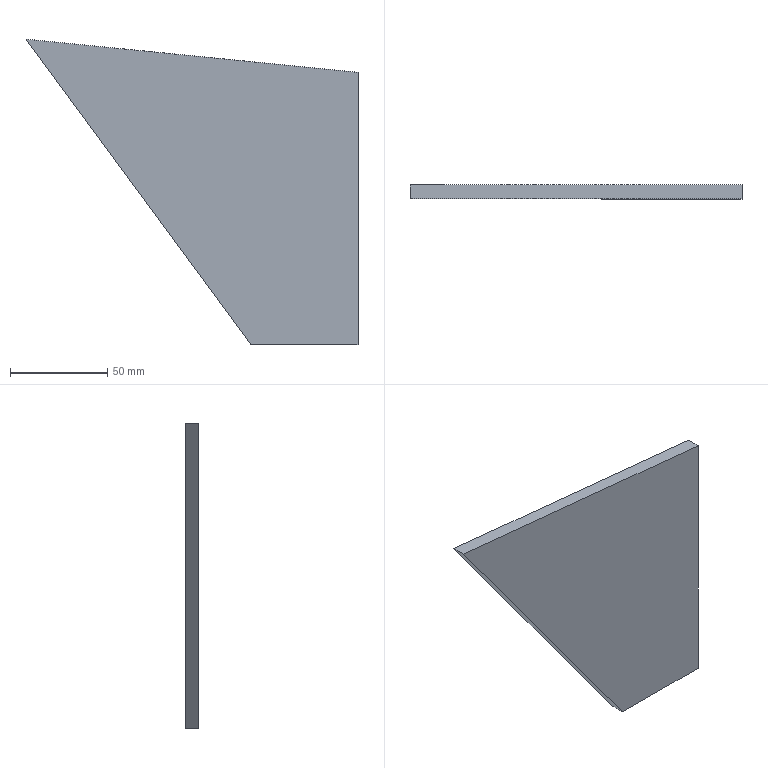Component | NX | TRIANGLE1_3 | 1 solid | 6 faces | box 170.57 x 7 x 157.02 mm | volume 113806 mm3 | plane 6
STEP:
#1=CARTESIAN_POINT('',(0.,0.,0.));
#2=DIRECTION('',(0.,0.,1.));
#3=DIRECTION('',(1.,0.,0.));
#4=AXIS2_PLACEMENT_3D('',#1,#2,#3);
#5=CARTESIAN_POINT('',(0.,142.,371.782));
#6=VERTEX_POINT('',#5);
#7=CARTESIAN_POINT('',(-115.568,142.,528.807));
#8=VERTEX_POINT('',#7);
#9=CARTESIAN_POINT('',(0.,142.,371.782));
#10=DIRECTION('',(-0.5928,0.,0.8054));
#11=VECTOR('',#10,1.);
#12=LINE('',#9,#11);
#13=CARTESIAN_POINT('',(0.,135.,371.782));
#14=DIRECTION('',(-0.8054,0.,-0.5928));
#15=DIRECTION('',(-0.5928,0.,0.8054));
#16=AXIS2_PLACEMENT_3D('',#13,#14,#15);
#17=PLANE('',#16);
#18=CARTESIAN_POINT('',(0.,7.));
#19=DIRECTION('',(1.,0.));
#20=VECTOR('',#19,1.);
#21=LINE('',#18,#20);
#22=(GEOMETRIC_REPRESENTATION_CONTEXT(2)PARAMETRIC_REPRESENTATION_CONTEXT()REPRESENTATION_CONTEXT('',''));
#23=DEFINITIONAL_REPRESENTATION('',(#21),#22);
#24=PCURVE('',#17,#23);
#25=CARTESIAN_POINT('',(-0.,142.,371.782));
#26=DIRECTION('',(0.,-1.,0.));
#27=DIRECTION('',(0.,0.,-1.));
#28=AXIS2_PLACEMENT_3D('',#25,#26,#27);
#29=PLANE('',#28);
#30=CARTESIAN_POINT('',(0.,0.));
#31=DIRECTION('',(-0.8054,-0.5928));
#32=VECTOR('',#31,1.);
#33=LINE('',#30,#32);
#34=(GEOMETRIC_REPRESENTATION_CONTEXT(2)PARAMETRIC_REPRESENTATION_CONTEXT()REPRESENTATION_CONTEXT('',''));
#35=DEFINITIONAL_REPRESENTATION('',(#33),#34);
#36=PCURVE('',#29,#35);
#37=SURFACE_CURVE('',#12,(#24,#36),.PCURVE_S1.);
#38=EDGE_CURVE('',#6,#8,#37,.T.);
#39=ORIENTED_EDGE('',*,*,#38,.F.);
#40=CARTESIAN_POINT('',(0.,135.,371.782));
#41=VERTEX_POINT('',#40);
#42=CARTESIAN_POINT('',(0.,135.,371.782));
#43=DIRECTION('',(0.,1.,0.));
#44=VECTOR('',#43,1.);
#45=LINE('',#42,#44);
#46=CARTESIAN_POINT('',(0.,0.));
#47=DIRECTION('',(0.,1.));
#48=VECTOR('',#47,1.);
#49=LINE('',#46,#48);
#50=(GEOMETRIC_REPRESENTATION_CONTEXT(2)PARAMETRIC_REPRESENTATION_CONTEXT()REPRESENTATION_CONTEXT('',''));
#51=DEFINITIONAL_REPRESENTATION('',(#49),#50);
#52=PCURVE('',#17,#51);
#53=CARTESIAN_POINT('',(55.,135.,371.782));
#54=DIRECTION('',(-0.,0.,-1.));
#55=DIRECTION('',(-1.,0.,0.));
#56=AXIS2_PLACEMENT_3D('',#53,#54,#55);
#57=PLANE('',#56);
#58=CARTESIAN_POINT('',(55.,0.));
#59=DIRECTION('',(0.,1.));
#60=VECTOR('',#59,1.);
#61=LINE('',#58,#60);
#62=(GEOMETRIC_REPRESENTATION_CONTEXT(2)PARAMETRIC_REPRESENTATION_CONTEXT()REPRESENTATION_CONTEXT('',''));
#63=DEFINITIONAL_REPRESENTATION('',(#61),#62);
#64=PCURVE('',#57,#63);
#65=SURFACE_CURVE('',#45,(#52,#64),.PCURVE_S1.);
#66=EDGE_CURVE('',#41,#6,#65,.T.);
#67=ORIENTED_EDGE('',*,*,#66,.F.);
#68=CARTESIAN_POINT('',(-115.568,135.,528.807));
#69=VERTEX_POINT('',#68);
#70=CARTESIAN_POINT('',(0.,135.,371.782));
#71=DIRECTION('',(-0.5928,0.,0.8054));
#72=VECTOR('',#71,1.);
#73=LINE('',#70,#72);
#74=CARTESIAN_POINT('',(0.,0.));
#75=DIRECTION('',(1.,0.));
#76=VECTOR('',#75,1.);
#77=LINE('',#74,#76);
#78=(GEOMETRIC_REPRESENTATION_CONTEXT(2)PARAMETRIC_REPRESENTATION_CONTEXT()REPRESENTATION_CONTEXT('',''));
#79=DEFINITIONAL_REPRESENTATION('',(#77),#78);
#80=PCURVE('',#17,#79);
#81=CARTESIAN_POINT('',(-0.,135.,371.782));
#82=DIRECTION('',(0.,-1.,0.));
#83=DIRECTION('',(0.,0.,-1.));
#84=AXIS2_PLACEMENT_3D('',#81,#82,#83);
#85=PLANE('',#84);
#86=CARTESIAN_POINT('',(0.,0.));
#87=DIRECTION('',(-0.8054,-0.5928));
#88=VECTOR('',#87,1.);
#89=LINE('',#86,#88);
#90=(GEOMETRIC_REPRESENTATION_CONTEXT(2)PARAMETRIC_REPRESENTATION_CONTEXT()REPRESENTATION_CONTEXT('',''));
#91=DEFINITIONAL_REPRESENTATION('',(#89),#90);
#92=PCURVE('',#85,#91);
#93=SURFACE_CURVE('',#73,(#80,#92),.PCURVE_S1.);
#94=EDGE_CURVE('',#41,#69,#93,.T.);
#95=ORIENTED_EDGE('',*,*,#94,.T.);
#96=CARTESIAN_POINT('',(-115.568,135.,528.807));
#97=DIRECTION('',(0.,1.,0.));
#98=VECTOR('',#97,1.);
#99=LINE('',#96,#98);
#100=CARTESIAN_POINT('',(194.969,0.));
#101=DIRECTION('',(0.,1.));
#102=VECTOR('',#101,1.);
#103=LINE('',#100,#102);
#104=(GEOMETRIC_REPRESENTATION_CONTEXT(2)PARAMETRIC_REPRESENTATION_CONTEXT()REPRESENTATION_CONTEXT('',''));
#105=DEFINITIONAL_REPRESENTATION('',(#103),#104);
#106=PCURVE('',#17,#105);
#107=CARTESIAN_POINT('',(-115.568,135.,528.807));
#108=DIRECTION('',(0.09932,0.,0.9951));
#109=DIRECTION('',(0.9951,0.,-0.09932));
#110=AXIS2_PLACEMENT_3D('',#107,#108,#109);
#111=PLANE('',#110);
#112=CARTESIAN_POINT('',(0.,0.));
#113=DIRECTION('',(0.,1.));
#114=VECTOR('',#113,1.);
#115=LINE('',#112,#114);
#116=(GEOMETRIC_REPRESENTATION_CONTEXT(2)PARAMETRIC_REPRESENTATION_CONTEXT()REPRESENTATION_CONTEXT('',''));
#117=DEFINITIONAL_REPRESENTATION('',(#115),#116);
#118=PCURVE('',#111,#117);
#119=SURFACE_CURVE('',#99,(#106,#118),.PCURVE_S1.);
#120=EDGE_CURVE('',#69,#8,#119,.T.);
#121=ORIENTED_EDGE('',*,*,#120,.T.);
#122=EDGE_LOOP('',(#39,#67,#95,#121));
#123=FACE_BOUND('',#122,.T.);
#124=ADVANCED_FACE('',(#123),#17,.T.);
#125=CARTESIAN_POINT('',(55.,142.,511.782));
#126=VERTEX_POINT('',#125);
#127=CARTESIAN_POINT('',(-115.568,142.,528.807));
#128=DIRECTION('',(0.9951,0.,-0.09932));
#129=VECTOR('',#128,1.);
#130=LINE('',#127,#129);
#131=CARTESIAN_POINT('',(0.,7.));
#132=DIRECTION('',(1.,0.));
#133=VECTOR('',#132,1.);
#134=LINE('',#131,#133);
#135=(GEOMETRIC_REPRESENTATION_CONTEXT(2)PARAMETRIC_REPRESENTATION_CONTEXT()REPRESENTATION_CONTEXT('',''));
#136=DEFINITIONAL_REPRESENTATION('',(#134),#135);
#137=PCURVE('',#111,#136);
#138=CARTESIAN_POINT('',(-157.025,-115.568));
#139=DIRECTION('',(0.09932,0.9951));
#140=VECTOR('',#139,1.);
#141=LINE('',#138,#140);
#142=(GEOMETRIC_REPRESENTATION_CONTEXT(2)PARAMETRIC_REPRESENTATION_CONTEXT()REPRESENTATION_CONTEXT('',''));
#143=DEFINITIONAL_REPRESENTATION('',(#141),#142);
#144=PCURVE('',#29,#143);
#145=SURFACE_CURVE('',#130,(#137,#144),.PCURVE_S1.);
#146=EDGE_CURVE('',#8,#126,#145,.T.);
#147=ORIENTED_EDGE('',*,*,#146,.F.);
#148=ORIENTED_EDGE('',*,*,#120,.F.);
#149=CARTESIAN_POINT('',(55.,135.,511.782));
#150=VERTEX_POINT('',#149);
#151=CARTESIAN_POINT('',(-115.568,135.,528.807));
#152=DIRECTION('',(0.9951,0.,-0.09932));
#153=VECTOR('',#152,1.);
#154=LINE('',#151,#153);
#155=CARTESIAN_POINT('',(0.,0.));
#156=DIRECTION('',(1.,0.));
#157=VECTOR('',#156,1.);
#158=LINE('',#155,#157);
#159=(GEOMETRIC_REPRESENTATION_CONTEXT(2)PARAMETRIC_REPRESENTATION_CONTEXT()REPRESENTATION_CONTEXT('',''));
#160=DEFINITIONAL_REPRESENTATION('',(#158),#159);
#161=PCURVE('',#111,#160);
#162=CARTESIAN_POINT('',(-157.025,-115.568));
#163=DIRECTION('',(0.09932,0.9951));
#164=VECTOR('',#163,1.);
#165=LINE('',#162,#164);
#166=(GEOMETRIC_REPRESENTATION_CONTEXT(2)PARAMETRIC_REPRESENTATION_CONTEXT()REPRESENTATION_CONTEXT('',''));
#167=DEFINITIONAL_REPRESENTATION('',(#165),#166);
#168=PCURVE('',#85,#167);
#169=SURFACE_CURVE('',#154,(#161,#168),.PCURVE_S1.);
#170=EDGE_CURVE('',#69,#150,#169,.T.);
#171=ORIENTED_EDGE('',*,*,#170,.T.);
#172=CARTESIAN_POINT('',(55.,135.,511.782));
#173=DIRECTION('',(0.,1.,0.));
#174=VECTOR('',#173,1.);
#175=LINE('',#172,#174);
#176=CARTESIAN_POINT('',(171.415,0.));
#177=DIRECTION('',(0.,1.));
#178=VECTOR('',#177,1.);
#179=LINE('',#176,#178);
#180=(GEOMETRIC_REPRESENTATION_CONTEXT(2)PARAMETRIC_REPRESENTATION_CONTEXT()REPRESENTATION_CONTEXT('',''));
#181=DEFINITIONAL_REPRESENTATION('',(#179),#180);
#182=PCURVE('',#111,#181);
#183=CARTESIAN_POINT('',(55.,135.,511.782));
#184=DIRECTION('',(1.,0.,0.));
#185=DIRECTION('',(0.,0.,-1.));
#186=AXIS2_PLACEMENT_3D('',#183,#184,#185);
#187=PLANE('',#186);
#188=CARTESIAN_POINT('',(0.,0.));
#189=DIRECTION('',(0.,1.));
#190=VECTOR('',#189,1.);
#191=LINE('',#188,#190);
#192=(GEOMETRIC_REPRESENTATION_CONTEXT(2)PARAMETRIC_REPRESENTATION_CONTEXT()REPRESENTATION_CONTEXT('',''));
#193=DEFINITIONAL_REPRESENTATION('',(#191),#192);
#194=PCURVE('',#187,#193);
#195=SURFACE_CURVE('',#175,(#182,#194),.PCURVE_S1.);
#196=EDGE_CURVE('',#150,#126,#195,.T.);
#197=ORIENTED_EDGE('',*,*,#196,.T.);
#198=EDGE_LOOP('',(#147,#148,#171,#197));
#199=FACE_BOUND('',#198,.T.);
#200=ADVANCED_FACE('',(#199),#111,.T.);
#201=CARTESIAN_POINT('',(55.,142.,371.782));
#202=VERTEX_POINT('',#201);
#203=CARTESIAN_POINT('',(55.,142.,511.782));
#204=DIRECTION('',(0.,0.,-1.));
#205=VECTOR('',#204,1.);
#206=LINE('',#203,#205);
#207=CARTESIAN_POINT('',(0.,7.));
#208=DIRECTION('',(1.,0.));
#209=VECTOR('',#208,1.);
#210=LINE('',#207,#209);
#211=(GEOMETRIC_REPRESENTATION_CONTEXT(2)PARAMETRIC_REPRESENTATION_CONTEXT()REPRESENTATION_CONTEXT('',''));
#212=DEFINITIONAL_REPRESENTATION('',(#210),#211);
#213=PCURVE('',#187,#212);
#214=CARTESIAN_POINT('',(-140.,55.));
#215=DIRECTION('',(1.,0.));
#216=VECTOR('',#215,1.);
#217=LINE('',#214,#216);
#218=(GEOMETRIC_REPRESENTATION_CONTEXT(2)PARAMETRIC_REPRESENTATION_CONTEXT()REPRESENTATION_CONTEXT('',''));
#219=DEFINITIONAL_REPRESENTATION('',(#217),#218);
#220=PCURVE('',#29,#219);
#221=SURFACE_CURVE('',#206,(#213,#220),.PCURVE_S1.);
#222=EDGE_CURVE('',#126,#202,#221,.T.);
#223=ORIENTED_EDGE('',*,*,#222,.F.);
#224=ORIENTED_EDGE('',*,*,#196,.F.);
#225=CARTESIAN_POINT('',(55.,135.,371.782));
#226=VERTEX_POINT('',#225);
#227=CARTESIAN_POINT('',(55.,135.,511.782));
#228=DIRECTION('',(0.,0.,-1.));
#229=VECTOR('',#228,1.);
#230=LINE('',#227,#229);
#231=CARTESIAN_POINT('',(0.,0.));
#232=DIRECTION('',(1.,0.));
#233=VECTOR('',#232,1.);
#234=LINE('',#231,#233);
#235=(GEOMETRIC_REPRESENTATION_CONTEXT(2)PARAMETRIC_REPRESENTATION_CONTEXT()REPRESENTATION_CONTEXT('',''));
#236=DEFINITIONAL_REPRESENTATION('',(#234),#235);
#237=PCURVE('',#187,#236);
#238=CARTESIAN_POINT('',(-140.,55.));
#239=DIRECTION('',(1.,0.));
#240=VECTOR('',#239,1.);
#241=LINE('',#238,#240);
#242=(GEOMETRIC_REPRESENTATION_CONTEXT(2)PARAMETRIC_REPRESENTATION_CONTEXT()REPRESENTATION_CONTEXT('',''));
#243=DEFINITIONAL_REPRESENTATION('',(#241),#242);
#244=PCURVE('',#85,#243);
#245=SURFACE_CURVE('',#230,(#237,#244),.PCURVE_S1.);
#246=EDGE_CURVE('',#150,#226,#245,.T.);
#247=ORIENTED_EDGE('',*,*,#246,.T.);
#248=CARTESIAN_POINT('',(55.,135.,371.782));
#249=DIRECTION('',(0.,1.,0.));
#250=VECTOR('',#249,1.);
#251=LINE('',#248,#250);
#252=CARTESIAN_POINT('',(140.,0.));
#253=DIRECTION('',(0.,1.));
#254=VECTOR('',#253,1.);
#255=LINE('',#252,#254);
#256=(GEOMETRIC_REPRESENTATION_CONTEXT(2)PARAMETRIC_REPRESENTATION_CONTEXT()REPRESENTATION_CONTEXT('',''));
#257=DEFINITIONAL_REPRESENTATION('',(#255),#256);
#258=PCURVE('',#187,#257);
#259=CARTESIAN_POINT('',(-0.,0.));
#260=DIRECTION('',(0.,1.));
#261=VECTOR('',#260,1.);
#262=LINE('',#259,#261);
#263=(GEOMETRIC_REPRESENTATION_CONTEXT(2)PARAMETRIC_REPRESENTATION_CONTEXT()REPRESENTATION_CONTEXT('',''));
#264=DEFINITIONAL_REPRESENTATION('',(#262),#263);
#265=PCURVE('',#57,#264);
#266=SURFACE_CURVE('',#251,(#258,#265),.PCURVE_S1.);
#267=EDGE_CURVE('',#226,#202,#266,.T.);
#268=ORIENTED_EDGE('',*,*,#267,.T.);
#269=EDGE_LOOP('',(#223,#224,#247,#268));
#270=FACE_BOUND('',#269,.T.);
#271=ADVANCED_FACE('',(#270),#187,.T.);
#272=CARTESIAN_POINT('',(55.,142.,371.782));
#273=DIRECTION('',(-1.,0.,0.));
#274=VECTOR('',#273,1.);
#275=LINE('',#272,#274);
#276=CARTESIAN_POINT('',(0.,7.));
#277=DIRECTION('',(1.,0.));
#278=VECTOR('',#277,1.);
#279=LINE('',#276,#278);
#280=(GEOMETRIC_REPRESENTATION_CONTEXT(2)PARAMETRIC_REPRESENTATION_CONTEXT()REPRESENTATION_CONTEXT('',''));
#281=DEFINITIONAL_REPRESENTATION('',(#279),#280);
#282=PCURVE('',#57,#281);
#283=CARTESIAN_POINT('',(0.,55.));
#284=DIRECTION('',(-0.,-1.));
#285=VECTOR('',#284,1.);
#286=LINE('',#283,#285);
#287=(GEOMETRIC_REPRESENTATION_CONTEXT(2)PARAMETRIC_REPRESENTATION_CONTEXT()REPRESENTATION_CONTEXT('',''));
#288=DEFINITIONAL_REPRESENTATION('',(#286),#287);
#289=PCURVE('',#29,#288);
#290=SURFACE_CURVE('',#275,(#282,#289),.PCURVE_S1.);
#291=EDGE_CURVE('',#202,#6,#290,.T.);
#292=ORIENTED_EDGE('',*,*,#291,.F.);
#293=ORIENTED_EDGE('',*,*,#267,.F.);
#294=CARTESIAN_POINT('',(55.,135.,371.782));
#295=DIRECTION('',(-1.,0.,0.));
#296=VECTOR('',#295,1.);
#297=LINE('',#294,#296);
#298=CARTESIAN_POINT('',(0.,0.));
#299=DIRECTION('',(1.,0.));
#300=VECTOR('',#299,1.);
#301=LINE('',#298,#300);
#302=(GEOMETRIC_REPRESENTATION_CONTEXT(2)PARAMETRIC_REPRESENTATION_CONTEXT()REPRESENTATION_CONTEXT('',''));
#303=DEFINITIONAL_REPRESENTATION('',(#301),#302);
#304=PCURVE('',#57,#303);
#305=CARTESIAN_POINT('',(0.,55.));
#306=DIRECTION('',(-0.,-1.));
#307=VECTOR('',#306,1.);
#308=LINE('',#305,#307);
#309=(GEOMETRIC_REPRESENTATION_CONTEXT(2)PARAMETRIC_REPRESENTATION_CONTEXT()REPRESENTATION_CONTEXT('',''));
#310=DEFINITIONAL_REPRESENTATION('',(#308),#309);
#311=PCURVE('',#85,#310);
#312=SURFACE_CURVE('',#297,(#304,#311),.PCURVE_S1.);
#313=EDGE_CURVE('',#226,#41,#312,.T.);
#314=ORIENTED_EDGE('',*,*,#313,.T.);
#315=ORIENTED_EDGE('',*,*,#66,.T.);
#316=EDGE_LOOP('',(#292,#293,#314,#315));
#317=FACE_BOUND('',#316,.T.);
#318=ADVANCED_FACE('',(#317),#57,.T.);
#319=ORIENTED_EDGE('',*,*,#94,.F.);
#320=ORIENTED_EDGE('',*,*,#313,.F.);
#321=ORIENTED_EDGE('',*,*,#246,.F.);
#322=ORIENTED_EDGE('',*,*,#170,.F.);
#323=EDGE_LOOP('',(#319,#320,#321,#322));
#324=FACE_BOUND('',#323,.T.);
#325=ADVANCED_FACE('',(#324),#85,.T.);
#326=ORIENTED_EDGE('',*,*,#38,.T.);
#327=ORIENTED_EDGE('',*,*,#146,.T.);
#328=ORIENTED_EDGE('',*,*,#222,.T.);
#329=ORIENTED_EDGE('',*,*,#291,.T.);
#330=EDGE_LOOP('',(#326,#327,#328,#329));
#331=FACE_BOUND('',#330,.T.);
#332=ADVANCED_FACE('',(#331),#29,.F.);
#333=CLOSED_SHELL('',(#124,#200,#271,#318,#325,#332));
#334=MANIFOLD_SOLID_BREP('',#333);
#335=(LENGTH_UNIT()NAMED_UNIT(*)SI_UNIT(.MILLI.,.METRE.));
#336=UNCERTAINTY_MEASURE_WITH_UNIT(LENGTH_MEASURE(0.0000001),#335,'','');
#337=(NAMED_UNIT(*)PLANE_ANGLE_UNIT()SI_UNIT($,.RADIAN.));
#338=(NAMED_UNIT(*)SI_UNIT($,.STERADIAN.)SOLID_ANGLE_UNIT());
#339=(GEOMETRIC_REPRESENTATION_CONTEXT(3)GLOBAL_UNCERTAINTY_ASSIGNED_CONTEXT((#336))GLOBAL_UNIT_ASSIGNED_CONTEXT((#335,#337,#338))REPRESENTATION_CONTEXT('',''));
#340=ADVANCED_BREP_SHAPE_REPRESENTATION('',(#4,#334),#339);